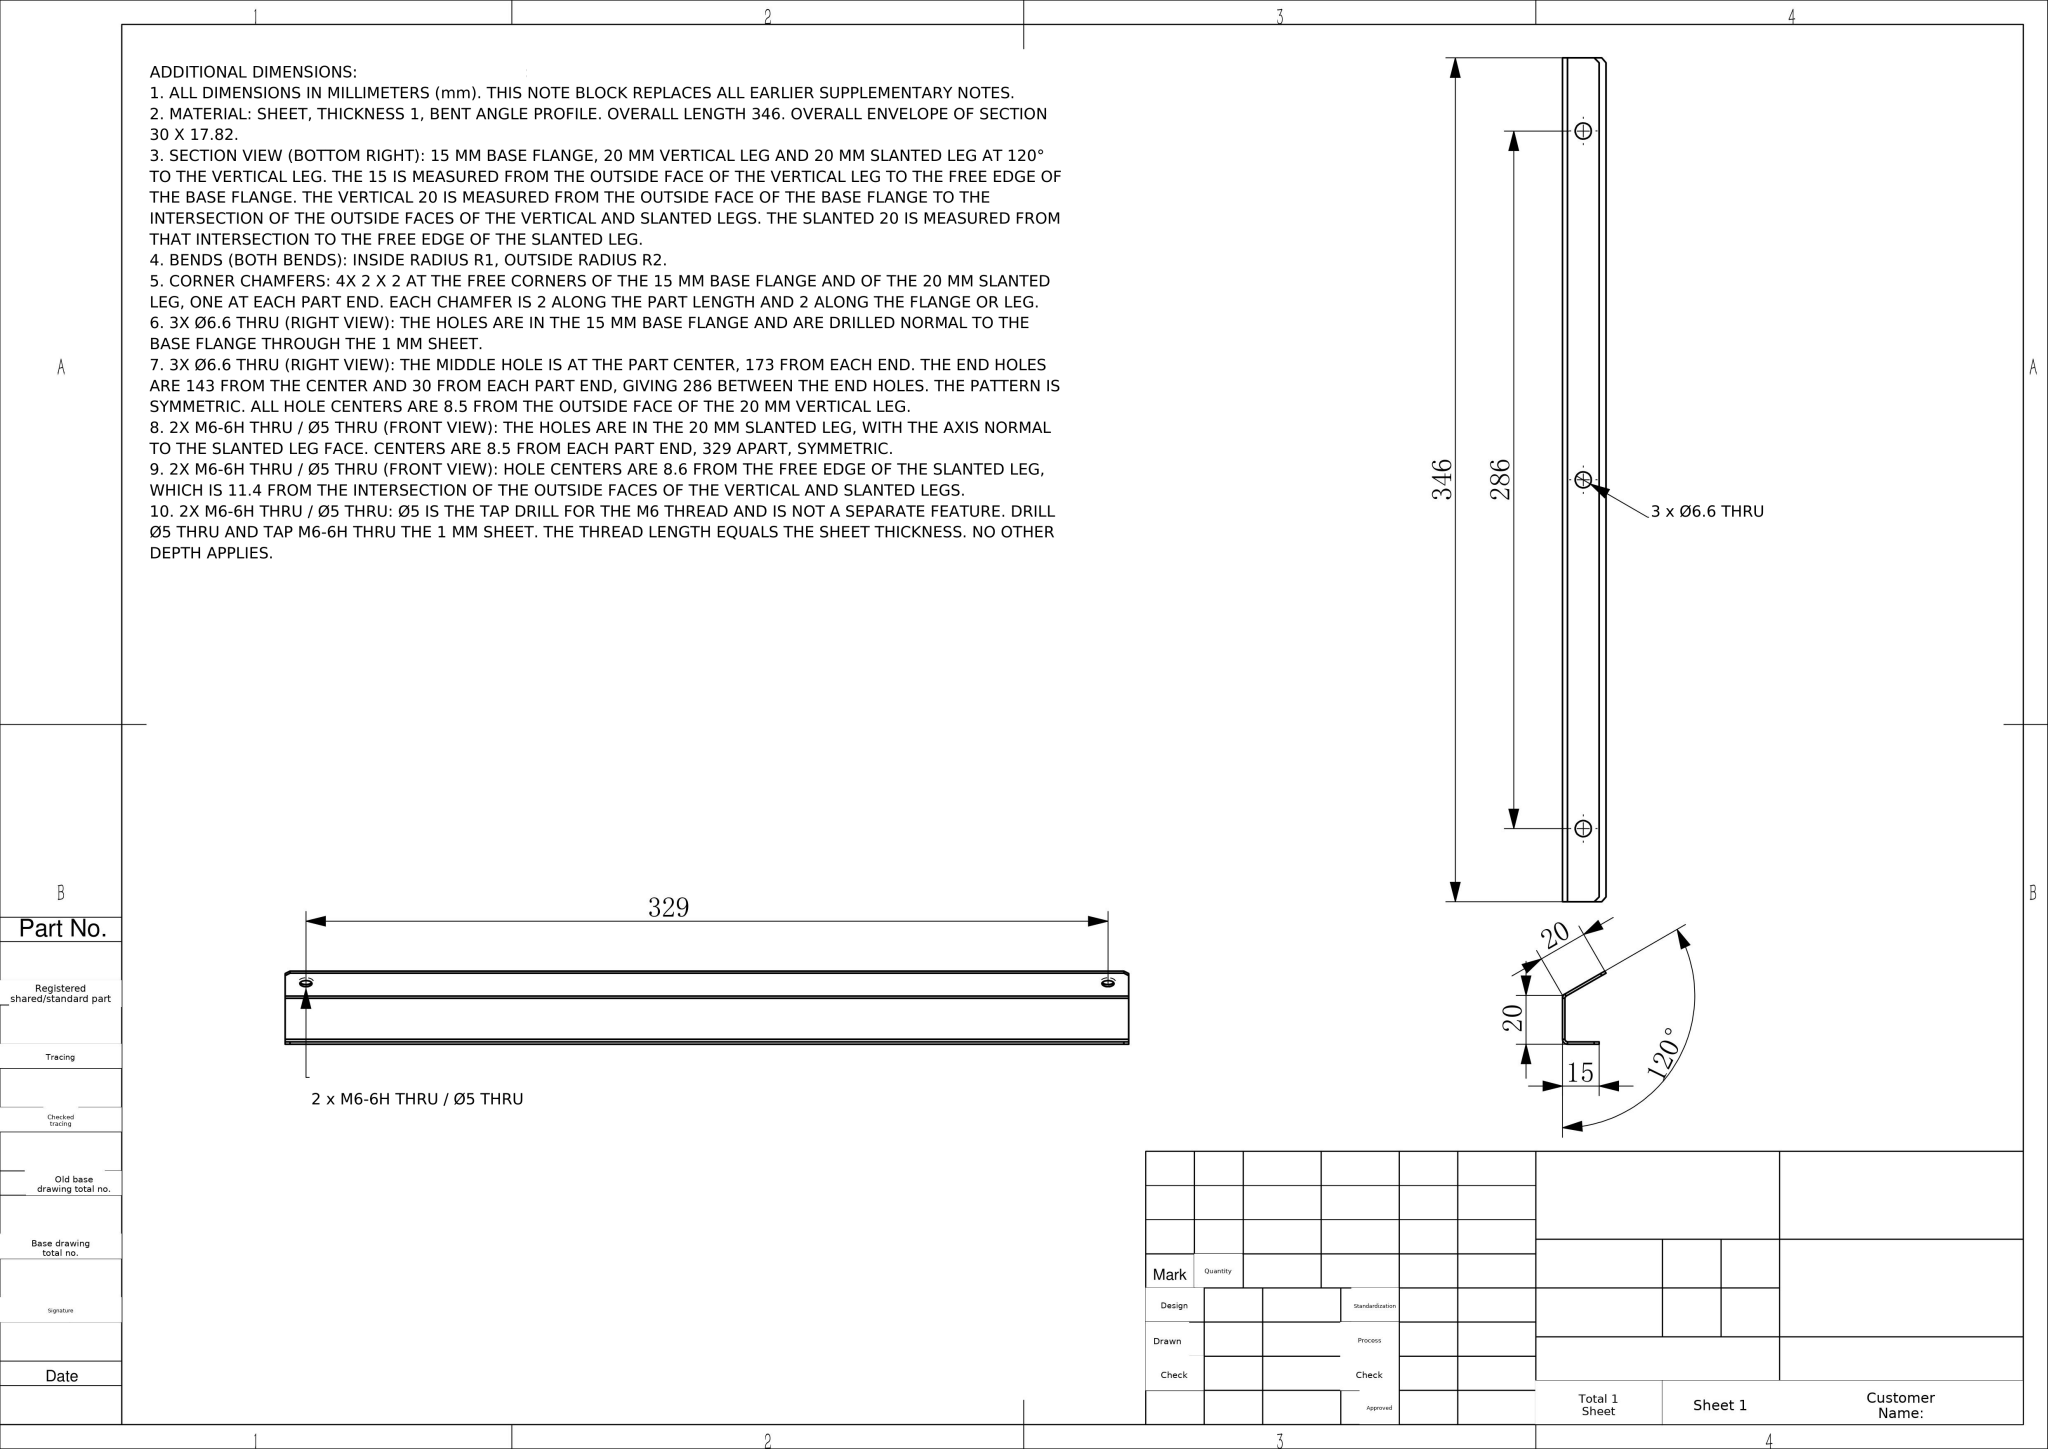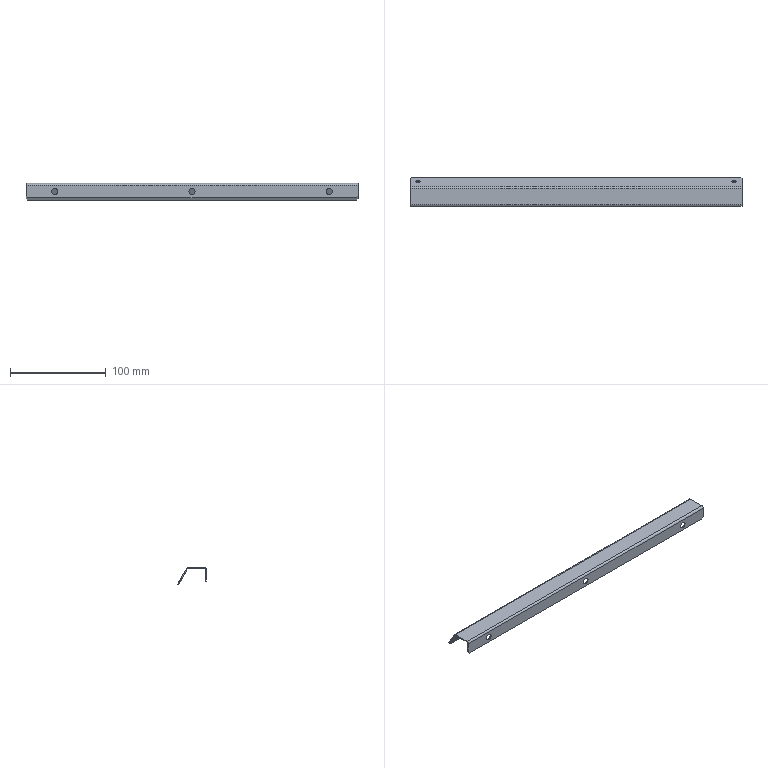Part | NX | mm | 1 solid | 36 faces | box 346 x 30 x 17.82 mm | volume 18056 mm3 | plane 22 | cylinder 14 | commonest cylinder face diameters 6.6 x6 5 x4 4 x2 2 x2